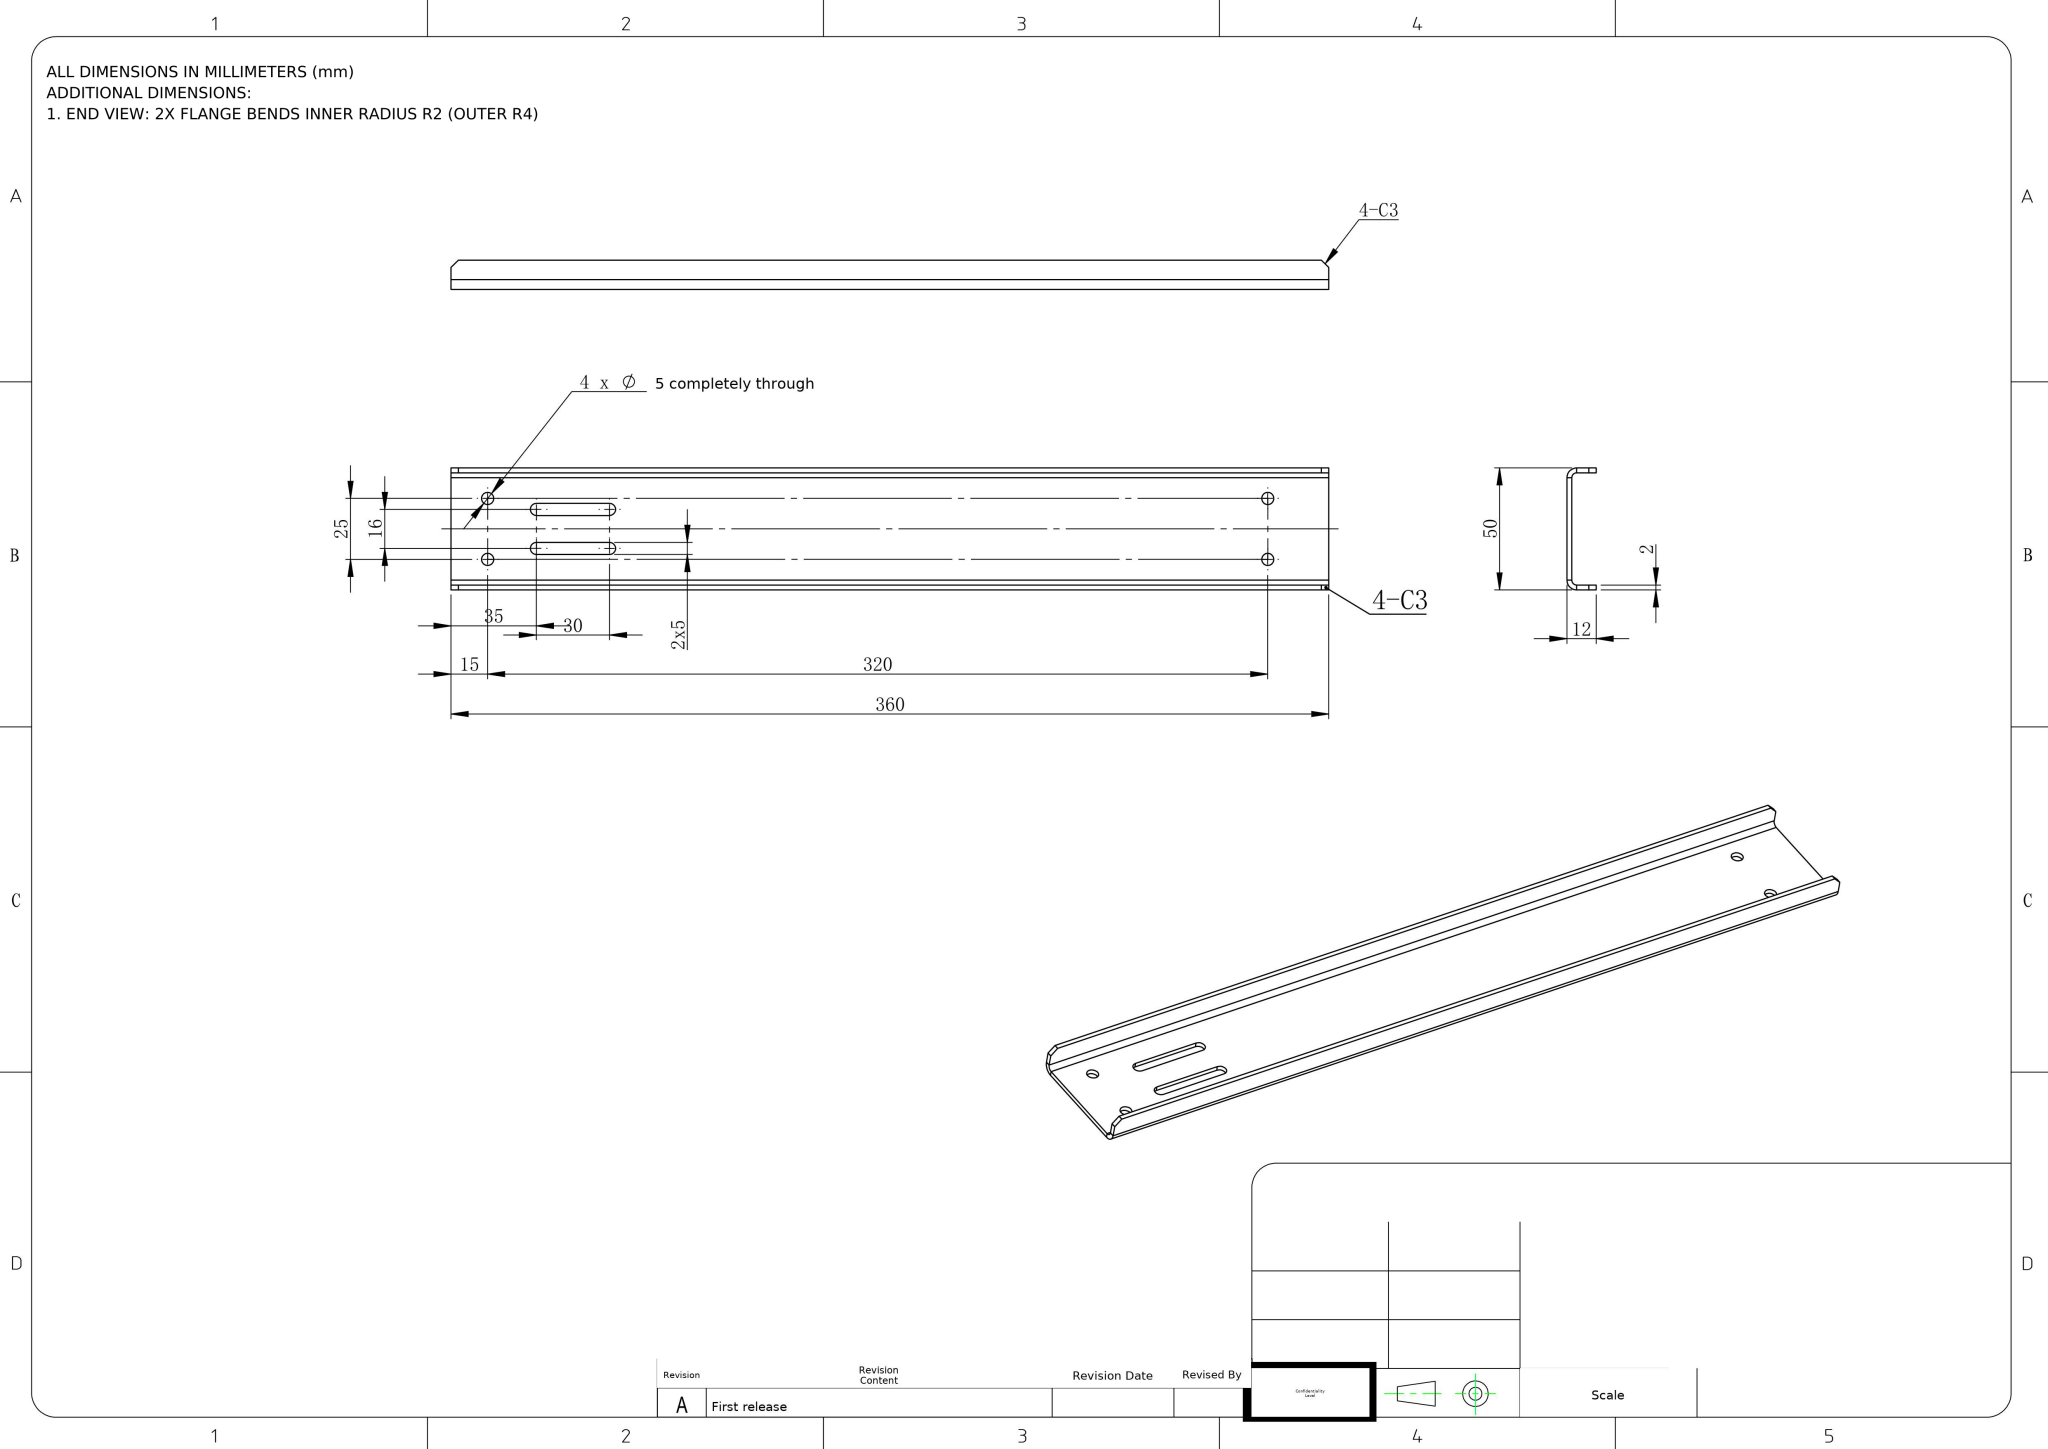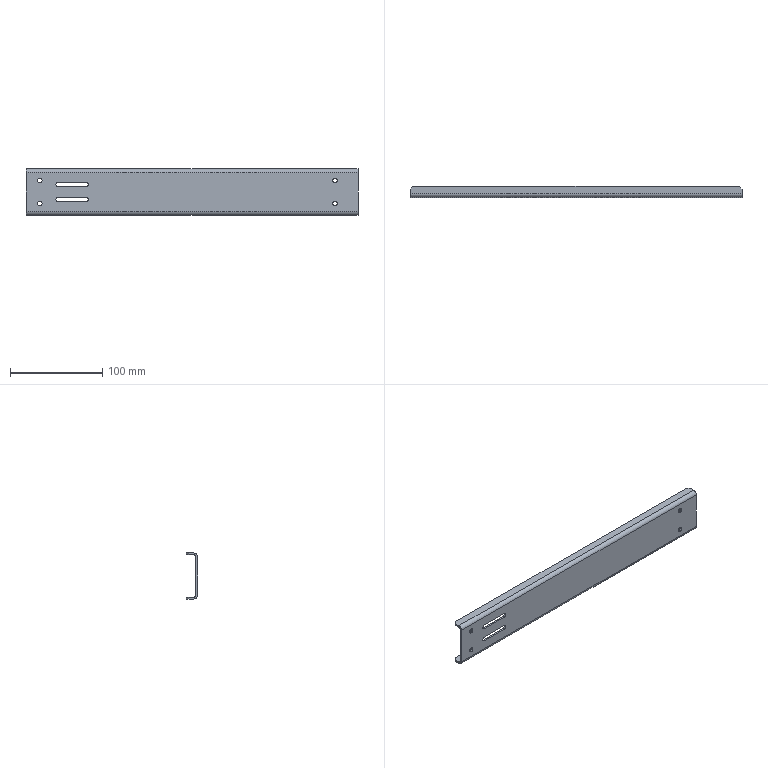Part | NX | mm | 1 solid | 42 faces | box 360 x 12 x 50 mm | volume 47674 mm3 | plane 26 | cylinder 16 | commonest cylinder face diameters 5 x12 8 x2 4 x2